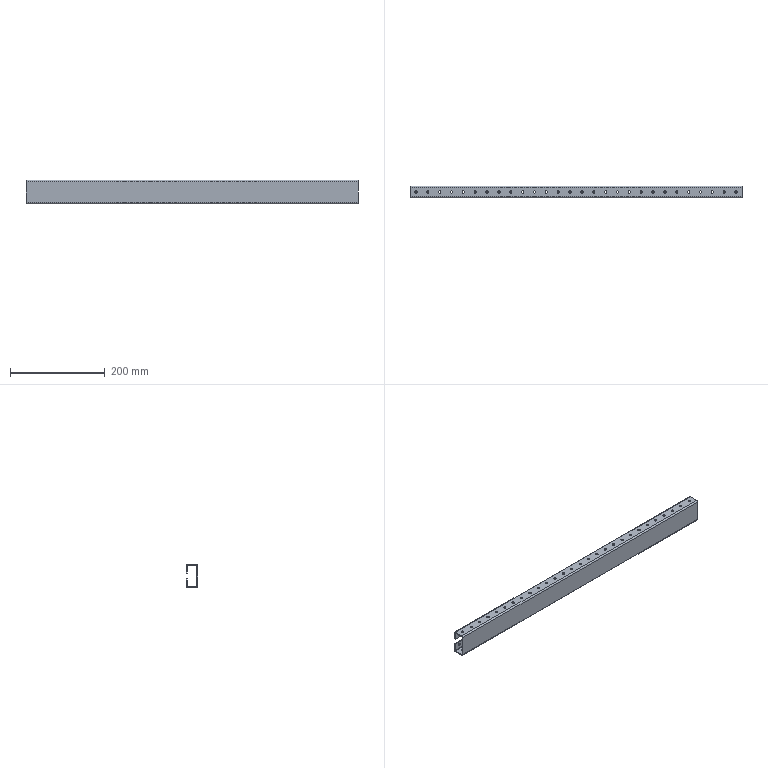Component | SolidWorks | Crossbeam(Item22)-2 | 1 solid | 262 faces | volume 172095 mm3 | cylinder 232 | plane 30 | commonest cylinder face diameters 5 x224 6 x4 2 x4 | material Plain Carbon Steel